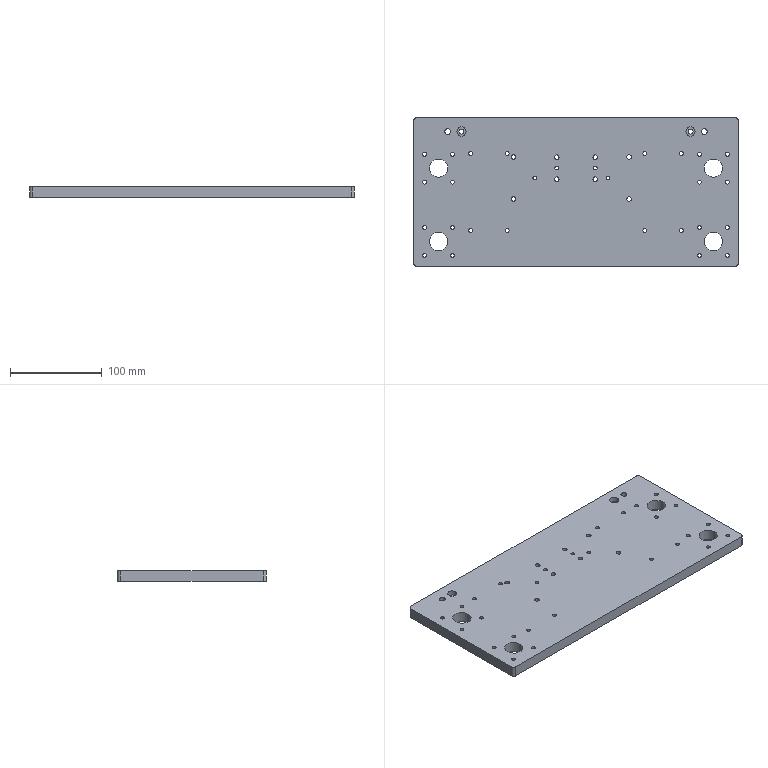Component | SolidWorks | J-005-1 | 1 solid | 126 faces | box 354 x 162 x 12 mm | volume 663054 mm3 | cylinder 108 | plane 10 | cone 8 | commonest cylinder face diameters 4.2 x56 5 x16 4 x8 20 x8 11 x4 6.6 x4 10 x4 5.5 x4 | material 45
build123d program:
from build123d import *

# Parameters (mm, degrees)
SKETCH1_W                                       = 354
SKETCH1_H                                       = 162
BOSS_EXTRUDE1_DEPTH                             = 12
SKETCH2_R                                       = 10
CUT_EXTRUDE4_DEPTH                              = 196.023
M5_TAPPED_HOLE1_D                               = 4.2
FILLET1_R                                       = 3
M5_TAPPED_HOLE2_D                               = 4.2
M6_TAPPED_HOLE1_D                               = 5
SIZE_MM_DOWEL_PIN_HOLE1_D                       = 4
M6_TAPPED_HOLE2_D                               = 5
SIZE_MM_DOWEL_PIN_HOLE2_D                       = 4
M5_TAPPED_HOLE3_D                               = 4.2
M5_TAPPED_HOLE3_DEPTH                           = 12.4
M5_TAPPED_HOLE3_TIP                             = 1.262
M5_HEX_SOCKET_HEAD_CAP_SCREW_CBORE1_D           = 5.5
M5_HEX_SOCKET_HEAD_CAP_SCREW_CBORE1_CBORE_D     = 10
M5_HEX_SOCKET_HEAD_CAP_SCREW_CBORE1_CBORE_DEPTH = 5.4
M6_HEX_SOCKET_HEAD_CAP_SCREW_CBORE1_D           = 6.6
M6_HEX_SOCKET_HEAD_CAP_SCREW_CBORE1_CBORE_D     = 11
M6_HEX_SOCKET_HEAD_CAP_SCREW_CBORE1_CBORE_DEPTH = 6.4


with BuildPart() as part:
    # Sketch1 → Boss-Extrude1 (new body)
    with BuildSketch(Plane.XY):
        Rectangle(SKETCH1_W, SKETCH1_H)
    extrude(amount=BOSS_EXTRUDE1_DEPTH)

    # Sketch2 → Cut-Extrude4 (cut, through all)
    with BuildSketch(Plane.XY.offset(12)):
        with Locations((-150, 26)):
            Circle(SKETCH2_R)
        with Locations((150, 26)):
            Circle(SKETCH2_R)
        with Locations((-150, -54)):
            Circle(SKETCH2_R)
        with Locations((150, -54)):
            Circle(SKETCH2_R)
    extrude(amount=-CUT_EXTRUDE4_DEPTH, mode=Mode.SUBTRACT)

    # M5 Tapped Hole1 (through all)
    with Locations(Plane.XY.offset(12)):
        with Locations((-165.203, 41.203), (-165.203, 10.797), (-134.797, 41.203), (-134.797, 10.797), (134.797, 41.203), (165.203, 41.203), (134.797, 10.797), (165.203, 10.797), (134.797, -38.797), (165.203, -38.797), (-165.203, -38.797), (-134.797, -38.797), (-165.203, -69.203), (-134.797, -69.203), (134.797, -69.203), (165.203, -69.203)):
            Hole(M5_TAPPED_HOLE1_D / 2)

    # Fillet1
    fillet1_edges = [part.edges().sort_by_distance(p)[0] for p in [
        (-177, 81, 6),
        (177, 81, 6),
        (177, -81, 6),
        (-177, -81, 6),
    ]]
    fillet(fillet1_edges, radius=FILLET1_R)

    # M5 Tapped Hole2 (through all)
    with Locations(Plane.XY.offset(12)):
        with Locations((-115, 42), (-115, -42), (-75, 42), (-75, -42), (75, 42), (75, -42), (115, 42), (115, -42)):
            Hole(M5_TAPPED_HOLE2_D / 2)

    # M6 Tapped Hole1 (through all)
    with Locations(Plane.XY.offset(12)):
        with Locations((-21, 14), (-21, 38), (21, 38), (21, 14)):
            Hole(M6_TAPPED_HOLE1_D / 2)

    # Size mm Dowel Pin Hole1 (through all)
    with Locations(Plane.XY.offset(12)):
        with Locations((-21, 26), (21, 26)):
            Hole(SIZE_MM_DOWEL_PIN_HOLE1_D / 2)

    # M6 Tapped Hole2 (through all)
    with Locations(Plane(origin=(0, 0, 0), x_dir=(-1, 0, 0), z_dir=(0, 0, -1))):
        with Locations((-58, 38.25), (68, 38.25), (-58, -7.75), (68, -7.75)):
            Hole(M6_TAPPED_HOLE2_D / 2)

    # Size mm Dowel Pin Hole2 (through all)
    with Locations(Plane(origin=(0, 0, 0), x_dir=(-1, 0, 0), z_dir=(0, 0, -1))):
        with Locations((-35, 15.25), (45, 15.25)):
            Hole(SIZE_MM_DOWEL_PIN_HOLE2_D / 2)

    # M5 Tapped Hole3
    with Locations(Plane(origin=(0, 81, 0), x_dir=(1, 0, 0), z_dir=(0, 1, 0))):
        with Locations((-150, -6), (-50, -6), (50, -6), (150, -6)):
            Hole(M5_TAPPED_HOLE3_D / 2, depth=M5_TAPPED_HOLE3_DEPTH)
            with Locations((0, 0, -(M5_TAPPED_HOLE3_DEPTH + M5_TAPPED_HOLE3_TIP / 2))):  # 118° drill point
                Cone(0, M5_TAPPED_HOLE3_D / 2, M5_TAPPED_HOLE3_TIP, mode=Mode.SUBTRACT)

    # M5 Hex Socket Head Cap Screw CBORE1 (through all)
    with Locations(Plane.XY.offset(12)):
        with Locations((125, 66), (-125, 66)):
            CounterBoreHole(M5_HEX_SOCKET_HEAD_CAP_SCREW_CBORE1_D / 2, M5_HEX_SOCKET_HEAD_CAP_SCREW_CBORE1_CBORE_D / 2, M5_HEX_SOCKET_HEAD_CAP_SCREW_CBORE1_CBORE_DEPTH)

    # M6 Hex Socket Head Cap Screw CBORE1 (through all)
    with Locations(Plane(origin=(0, 0, 0), x_dir=(-1, 0, 0), z_dir=(0, 0, -1))):
        with Locations((-140, 66), (140, 66)):
            CounterBoreHole(M6_HEX_SOCKET_HEAD_CAP_SCREW_CBORE1_D / 2, M6_HEX_SOCKET_HEAD_CAP_SCREW_CBORE1_CBORE_D / 2, M6_HEX_SOCKET_HEAD_CAP_SCREW_CBORE1_CBORE_DEPTH)


solid = part.part

# Placed as in the assembly
solid = solid.moved(Location((220.325, 177.019, 264.731), (0, 0, 0)))